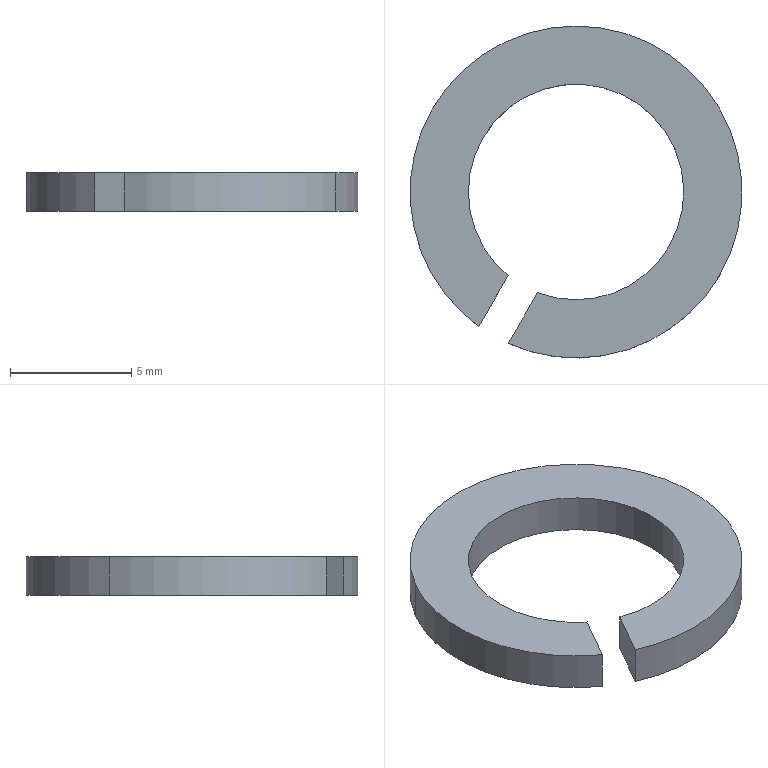Component | NX | SADDLE_SPRING_WASHER_8_4 | 1 solid | 10 faces | box 13.68 x 13.68 x 1.6 mm | volume 131 mm3 | cylinder 6 | plane 4 | commonest cylinder face diameters 8.88 x3 13.68 x3
STEP:
#1=CARTESIAN_POINT('',(0.,0.,0.));
#2=DIRECTION('',(0.,0.,1.));
#3=DIRECTION('',(1.,0.,0.));
#4=AXIS2_PLACEMENT_3D('',#1,#2,#3);
#5=CARTESIAN_POINT('',(-101.706,67.22,-42.5));
#6=VERTEX_POINT('',#5);
#7=CARTESIAN_POINT('',(-101.706,67.22,-40.9));
#8=VERTEX_POINT('',#7);
#9=CARTESIAN_POINT('',(-101.706,67.22,-41.7));
#10=DIRECTION('',(0.,0.,1.));
#11=VECTOR('',#10,1.);
#12=LINE('',#9,#11);
#13=CARTESIAN_POINT('',(-97.861,65.,-41.7));
#14=DIRECTION('',(0.,0.,1.));
#15=DIRECTION('',(0.866,-0.5,0.));
#16=AXIS2_PLACEMENT_3D('',#13,#14,#15);
#17=CYLINDRICAL_SURFACE('',#16,4.44);
#18=CARTESIAN_POINT('',(3.142,0.));
#19=DIRECTION('',(0.,1.));
#20=VECTOR('',#19,1.);
#21=LINE('',#18,#20);
#22=(GEOMETRIC_REPRESENTATION_CONTEXT(2)PARAMETRIC_REPRESENTATION_CONTEXT()REPRESENTATION_CONTEXT('',''));
#23=DEFINITIONAL_REPRESENTATION('',(#21),#22);
#24=PCURVE('',#17,#23);
#25=CARTESIAN_POINT('',(-97.861,65.,-41.7));
#26=DIRECTION('',(0.,0.,1.));
#27=DIRECTION('',(0.866,-0.5,0.));
#28=AXIS2_PLACEMENT_3D('',#25,#26,#27);
#29=CYLINDRICAL_SURFACE('',#28,4.44);
#30=CARTESIAN_POINT('',(3.142,0.));
#31=DIRECTION('',(0.,1.));
#32=VECTOR('',#31,1.);
#33=LINE('',#30,#32);
#34=(GEOMETRIC_REPRESENTATION_CONTEXT(2)PARAMETRIC_REPRESENTATION_CONTEXT()REPRESENTATION_CONTEXT('',''));
#35=DEFINITIONAL_REPRESENTATION('',(#33),#34);
#36=PCURVE('',#29,#35);
#37=SURFACE_CURVE('',#12,(#24,#36),.PCURVE_S1.);
#38=EDGE_CURVE('',#6,#8,#37,.T.);
#39=ORIENTED_EDGE('',*,*,#38,.T.);
#40=CARTESIAN_POINT('',(-94.016,62.78,-40.9));
#41=VERTEX_POINT('',#40);
#42=CARTESIAN_POINT('',(-97.861,65.,-40.9));
#43=DIRECTION('',(0.,0.,1.));
#44=DIRECTION('',(-0.866,0.5,0.));
#45=AXIS2_PLACEMENT_3D('',#42,#43,#44);
#46=CIRCLE('',#45,4.44);
#47=CARTESIAN_POINT('',(-3.142,0.8));
#48=DIRECTION('',(1.,0.));
#49=VECTOR('',#48,1.);
#50=LINE('',#47,#49);
#51=(GEOMETRIC_REPRESENTATION_CONTEXT(2)PARAMETRIC_REPRESENTATION_CONTEXT()REPRESENTATION_CONTEXT('',''));
#52=DEFINITIONAL_REPRESENTATION('',(#50),#51);
#53=PCURVE('',#17,#52);
#54=CARTESIAN_POINT('',(-97.861,65.,-40.9));
#55=DIRECTION('',(0.,0.,1.));
#56=DIRECTION('',(0.866,-0.5,0.));
#57=AXIS2_PLACEMENT_3D('',#54,#55,#56);
#58=PLANE('',#57);
#59=CARTESIAN_POINT('',(0.,0.));
#60=DIRECTION('',(-1.,0.));
#61=AXIS2_PLACEMENT_2D('',#59,#60);
#62=CIRCLE('',#61,4.44);
#63=(GEOMETRIC_REPRESENTATION_CONTEXT(2)PARAMETRIC_REPRESENTATION_CONTEXT()REPRESENTATION_CONTEXT('',''));
#64=DEFINITIONAL_REPRESENTATION('',(#62),#63);
#65=PCURVE('',#58,#64);
#66=SURFACE_CURVE('',#46,(#53,#65),.PCURVE_S1.);
#67=EDGE_CURVE('',#41,#8,#66,.T.);
#68=ORIENTED_EDGE('',*,*,#67,.F.);
#69=CARTESIAN_POINT('',(-94.016,62.78,-42.5));
#70=VERTEX_POINT('',#69);
#71=CARTESIAN_POINT('',(-94.016,62.78,-41.7));
#72=DIRECTION('',(0.,0.,1.));
#73=VECTOR('',#72,1.);
#74=LINE('',#71,#73);
#75=CARTESIAN_POINT('',(0.,0.));
#76=DIRECTION('',(0.,1.));
#77=VECTOR('',#76,1.);
#78=LINE('',#75,#77);
#79=(GEOMETRIC_REPRESENTATION_CONTEXT(2)PARAMETRIC_REPRESENTATION_CONTEXT()REPRESENTATION_CONTEXT('',''));
#80=DEFINITIONAL_REPRESENTATION('',(#78),#79);
#81=PCURVE('',#17,#80);
#82=CARTESIAN_POINT('',(-97.861,65.,-41.7));
#83=DIRECTION('',(0.,0.,1.));
#84=DIRECTION('',(0.866,-0.5,0.));
#85=AXIS2_PLACEMENT_3D('',#82,#83,#84);
#86=CYLINDRICAL_SURFACE('',#85,4.44);
#87=CARTESIAN_POINT('',(6.283,0.));
#88=DIRECTION('',(0.,1.));
#89=VECTOR('',#88,1.);
#90=LINE('',#87,#89);
#91=(GEOMETRIC_REPRESENTATION_CONTEXT(2)PARAMETRIC_REPRESENTATION_CONTEXT()REPRESENTATION_CONTEXT('',''));
#92=DEFINITIONAL_REPRESENTATION('',(#90),#91);
#93=PCURVE('',#86,#92);
#94=SURFACE_CURVE('',#74,(#81,#93),.PCURVE_S1.);
#95=EDGE_CURVE('',#70,#41,#94,.T.);
#96=ORIENTED_EDGE('',*,*,#95,.F.);
#97=CARTESIAN_POINT('',(-97.861,65.,-42.5));
#98=DIRECTION('',(0.,0.,1.));
#99=DIRECTION('',(-0.866,0.5,0.));
#100=AXIS2_PLACEMENT_3D('',#97,#98,#99);
#101=CIRCLE('',#100,4.44);
#102=CARTESIAN_POINT('',(-3.142,-0.8));
#103=DIRECTION('',(1.,0.));
#104=VECTOR('',#103,1.);
#105=LINE('',#102,#104);
#106=(GEOMETRIC_REPRESENTATION_CONTEXT(2)PARAMETRIC_REPRESENTATION_CONTEXT()REPRESENTATION_CONTEXT('',''));
#107=DEFINITIONAL_REPRESENTATION('',(#105),#106);
#108=PCURVE('',#17,#107);
#109=CARTESIAN_POINT('',(-97.861,65.,-42.5));
#110=DIRECTION('',(0.,0.,1.));
#111=DIRECTION('',(0.866,-0.5,0.));
#112=AXIS2_PLACEMENT_3D('',#109,#110,#111);
#113=PLANE('',#112);
#114=CARTESIAN_POINT('',(0.,0.));
#115=DIRECTION('',(-1.,0.));
#116=AXIS2_PLACEMENT_2D('',#114,#115);
#117=CIRCLE('',#116,4.44);
#118=(GEOMETRIC_REPRESENTATION_CONTEXT(2)PARAMETRIC_REPRESENTATION_CONTEXT()REPRESENTATION_CONTEXT('',''));
#119=DEFINITIONAL_REPRESENTATION('',(#117),#118);
#120=PCURVE('',#113,#119);
#121=SURFACE_CURVE('',#101,(#108,#120),.PCURVE_S1.);
#122=EDGE_CURVE('',#70,#6,#121,.T.);
#123=ORIENTED_EDGE('',*,*,#122,.T.);
#124=EDGE_LOOP('',(#39,#68,#96,#123));
#125=FACE_BOUND('',#124,.F.);
#126=ADVANCED_FACE('',(#125),#17,.F.);
#127=CARTESIAN_POINT('',(-100.659,61.553,-40.9));
#128=VERTEX_POINT('',#127);
#129=CARTESIAN_POINT('',(-100.659,61.553,-42.5));
#130=VERTEX_POINT('',#129);
#131=CARTESIAN_POINT('',(-100.659,61.553,-41.7));
#132=DIRECTION('',(0.,0.,-1.));
#133=VECTOR('',#132,1.);
#134=LINE('',#131,#133);
#135=CARTESIAN_POINT('',(4.554,0.));
#136=DIRECTION('',(0.,-1.));
#137=VECTOR('',#136,1.);
#138=LINE('',#135,#137);
#139=(GEOMETRIC_REPRESENTATION_CONTEXT(2)PARAMETRIC_REPRESENTATION_CONTEXT()REPRESENTATION_CONTEXT('',''));
#140=DEFINITIONAL_REPRESENTATION('',(#138),#139);
#141=PCURVE('',#29,#140);
#142=CARTESIAN_POINT('',(-100.609,61.641,-40.9));
#143=DIRECTION('',(-0.866,0.5,0.));
#144=DIRECTION('',(-0.5,-0.866,0.));
#145=AXIS2_PLACEMENT_3D('',#142,#143,#144);
#146=PLANE('',#145);
#147=CARTESIAN_POINT('',(0.1013,-0.8));
#148=DIRECTION('',(0.,-1.));
#149=VECTOR('',#148,1.);
#150=LINE('',#147,#149);
#151=(GEOMETRIC_REPRESENTATION_CONTEXT(2)PARAMETRIC_REPRESENTATION_CONTEXT()REPRESENTATION_CONTEXT('',''));
#152=DEFINITIONAL_REPRESENTATION('',(#150),#151);
#153=PCURVE('',#146,#152);
#154=SURFACE_CURVE('',#134,(#141,#153),.PCURVE_S1.);
#155=EDGE_CURVE('',#128,#130,#154,.T.);
#156=ORIENTED_EDGE('',*,*,#155,.F.);
#157=CARTESIAN_POINT('',(-97.861,65.,-40.9));
#158=DIRECTION('',(0.,0.,1.));
#159=DIRECTION('',(-0.866,0.5,0.));
#160=AXIS2_PLACEMENT_3D('',#157,#158,#159);
#161=CIRCLE('',#160,4.44);
#162=CARTESIAN_POINT('',(3.142,0.8));
#163=DIRECTION('',(1.,0.));
#164=VECTOR('',#163,1.);
#165=LINE('',#162,#164);
#166=(GEOMETRIC_REPRESENTATION_CONTEXT(2)PARAMETRIC_REPRESENTATION_CONTEXT()REPRESENTATION_CONTEXT('',''));
#167=DEFINITIONAL_REPRESENTATION('',(#165),#166);
#168=PCURVE('',#29,#167);
#169=CARTESIAN_POINT('',(0.,0.));
#170=DIRECTION('',(-1.,0.));
#171=AXIS2_PLACEMENT_2D('',#169,#170);
#172=CIRCLE('',#171,4.44);
#173=(GEOMETRIC_REPRESENTATION_CONTEXT(2)PARAMETRIC_REPRESENTATION_CONTEXT()REPRESENTATION_CONTEXT('',''));
#174=DEFINITIONAL_REPRESENTATION('',(#172),#173);
#175=PCURVE('',#58,#174);
#176=SURFACE_CURVE('',#161,(#168,#175),.PCURVE_S1.);
#177=EDGE_CURVE('',#8,#128,#176,.T.);
#178=ORIENTED_EDGE('',*,*,#177,.F.);
#179=ORIENTED_EDGE('',*,*,#38,.F.);
#180=CARTESIAN_POINT('',(-97.861,65.,-42.5));
#181=DIRECTION('',(0.,0.,1.));
#182=DIRECTION('',(-0.866,0.5,0.));
#183=AXIS2_PLACEMENT_3D('',#180,#181,#182);
#184=CIRCLE('',#183,4.44);
#185=CARTESIAN_POINT('',(3.142,-0.8));
#186=DIRECTION('',(1.,0.));
#187=VECTOR('',#186,1.);
#188=LINE('',#185,#187);
#189=(GEOMETRIC_REPRESENTATION_CONTEXT(2)PARAMETRIC_REPRESENTATION_CONTEXT()REPRESENTATION_CONTEXT('',''));
#190=DEFINITIONAL_REPRESENTATION('',(#188),#189);
#191=PCURVE('',#29,#190);
#192=CARTESIAN_POINT('',(0.,0.));
#193=DIRECTION('',(-1.,0.));
#194=AXIS2_PLACEMENT_2D('',#192,#193);
#195=CIRCLE('',#194,4.44);
#196=(GEOMETRIC_REPRESENTATION_CONTEXT(2)PARAMETRIC_REPRESENTATION_CONTEXT()REPRESENTATION_CONTEXT('',''));
#197=DEFINITIONAL_REPRESENTATION('',(#195),#196);
#198=PCURVE('',#113,#197);
#199=SURFACE_CURVE('',#184,(#191,#198),.PCURVE_S1.);
#200=EDGE_CURVE('',#6,#130,#199,.T.);
#201=ORIENTED_EDGE('',*,*,#200,.T.);
#202=EDGE_LOOP('',(#156,#178,#179,#201));
#203=FACE_BOUND('',#202,.F.);
#204=ADVANCED_FACE('',(#203),#29,.F.);
#205=CARTESIAN_POINT('',(-100.657,58.757,-42.5));
#206=VERTEX_POINT('',#205);
#207=CARTESIAN_POINT('',(-91.937,61.58,-42.5));
#208=VERTEX_POINT('',#207);
#209=CARTESIAN_POINT('',(-97.861,65.,-42.5));
#210=DIRECTION('',(0.,0.,1.));
#211=DIRECTION('',(-0.866,0.5,0.));
#212=AXIS2_PLACEMENT_3D('',#209,#210,#211);
#213=CIRCLE('',#212,6.84);
#214=CARTESIAN_POINT('',(-97.861,65.,-41.7));
#215=DIRECTION('',(0.,0.,1.));
#216=DIRECTION('',(0.866,-0.5,0.));
#217=AXIS2_PLACEMENT_3D('',#214,#215,#216);
#218=CYLINDRICAL_SURFACE('',#217,6.84);
#219=CARTESIAN_POINT('',(3.142,-0.8));
#220=DIRECTION('',(1.,0.));
#221=VECTOR('',#220,1.);
#222=LINE('',#219,#221);
#223=(GEOMETRIC_REPRESENTATION_CONTEXT(2)PARAMETRIC_REPRESENTATION_CONTEXT()REPRESENTATION_CONTEXT('',''));
#224=DEFINITIONAL_REPRESENTATION('',(#222),#223);
#225=PCURVE('',#218,#224);
#226=CARTESIAN_POINT('',(0.,0.));
#227=DIRECTION('',(-1.,0.));
#228=AXIS2_PLACEMENT_2D('',#226,#227);
#229=CIRCLE('',#228,6.84);
#230=(GEOMETRIC_REPRESENTATION_CONTEXT(2)PARAMETRIC_REPRESENTATION_CONTEXT()REPRESENTATION_CONTEXT('',''));
#231=DEFINITIONAL_REPRESENTATION('',(#229),#230);
#232=PCURVE('',#113,#231);
#233=SURFACE_CURVE('',#213,(#225,#232),.PCURVE_S1.);
#234=EDGE_CURVE('',#206,#208,#233,.T.);
#235=ORIENTED_EDGE('',*,*,#234,.T.);
#236=CARTESIAN_POINT('',(-91.937,61.58,-40.9));
#237=VERTEX_POINT('',#236);
#238=CARTESIAN_POINT('',(-91.937,61.58,-41.7));
#239=DIRECTION('',(0.,0.,1.));
#240=VECTOR('',#239,1.);
#241=LINE('',#238,#240);
#242=CARTESIAN_POINT('',(6.283,0.));
#243=DIRECTION('',(0.,1.));
#244=VECTOR('',#243,1.);
#245=LINE('',#242,#244);
#246=(GEOMETRIC_REPRESENTATION_CONTEXT(2)PARAMETRIC_REPRESENTATION_CONTEXT()REPRESENTATION_CONTEXT('',''));
#247=DEFINITIONAL_REPRESENTATION('',(#245),#246);
#248=PCURVE('',#218,#247);
#249=CARTESIAN_POINT('',(-97.861,65.,-41.7));
#250=DIRECTION('',(0.,0.,1.));
#251=DIRECTION('',(0.866,-0.5,0.));
#252=AXIS2_PLACEMENT_3D('',#249,#250,#251);
#253=CYLINDRICAL_SURFACE('',#252,6.84);
#254=CARTESIAN_POINT('',(0.,0.));
#255=DIRECTION('',(0.,1.));
#256=VECTOR('',#255,1.);
#257=LINE('',#254,#256);
#258=(GEOMETRIC_REPRESENTATION_CONTEXT(2)PARAMETRIC_REPRESENTATION_CONTEXT()REPRESENTATION_CONTEXT('',''));
#259=DEFINITIONAL_REPRESENTATION('',(#257),#258);
#260=PCURVE('',#253,#259);
#261=SURFACE_CURVE('',#241,(#248,#260),.PCURVE_S1.);
#262=EDGE_CURVE('',#208,#237,#261,.T.);
#263=ORIENTED_EDGE('',*,*,#262,.T.);
#264=CARTESIAN_POINT('',(-100.657,58.757,-40.9));
#265=VERTEX_POINT('',#264);
#266=CARTESIAN_POINT('',(-97.861,65.,-40.9));
#267=DIRECTION('',(0.,0.,1.));
#268=DIRECTION('',(-0.866,0.5,0.));
#269=AXIS2_PLACEMENT_3D('',#266,#267,#268);
#270=CIRCLE('',#269,6.84);
#271=CARTESIAN_POINT('',(3.142,0.8));
#272=DIRECTION('',(1.,0.));
#273=VECTOR('',#272,1.);
#274=LINE('',#271,#273);
#275=(GEOMETRIC_REPRESENTATION_CONTEXT(2)PARAMETRIC_REPRESENTATION_CONTEXT()REPRESENTATION_CONTEXT('',''));
#276=DEFINITIONAL_REPRESENTATION('',(#274),#275);
#277=PCURVE('',#218,#276);
#278=CARTESIAN_POINT('',(0.,0.));
#279=DIRECTION('',(-1.,0.));
#280=AXIS2_PLACEMENT_2D('',#278,#279);
#281=CIRCLE('',#280,6.84);
#282=(GEOMETRIC_REPRESENTATION_CONTEXT(2)PARAMETRIC_REPRESENTATION_CONTEXT()REPRESENTATION_CONTEXT('',''));
#283=DEFINITIONAL_REPRESENTATION('',(#281),#282);
#284=PCURVE('',#58,#283);
#285=SURFACE_CURVE('',#270,(#277,#284),.PCURVE_S1.);
#286=EDGE_CURVE('',#265,#237,#285,.T.);
#287=ORIENTED_EDGE('',*,*,#286,.F.);
#288=CARTESIAN_POINT('',(-100.657,58.757,-41.7));
#289=DIRECTION('',(0.,0.,-1.));
#290=VECTOR('',#289,1.);
#291=LINE('',#288,#290);
#292=CARTESIAN_POINT('',(4.815,0.));
#293=DIRECTION('',(0.,-1.));
#294=VECTOR('',#293,1.);
#295=LINE('',#292,#294);
#296=(GEOMETRIC_REPRESENTATION_CONTEXT(2)PARAMETRIC_REPRESENTATION_CONTEXT()REPRESENTATION_CONTEXT('',''));
#297=DEFINITIONAL_REPRESENTATION('',(#295),#296);
#298=PCURVE('',#218,#297);
#299=CARTESIAN_POINT('',(-99.396,60.941,-40.9));
#300=DIRECTION('',(0.866,-0.5,0.));
#301=DIRECTION('',(0.5,0.866,0.));
#302=AXIS2_PLACEMENT_3D('',#299,#300,#301);
#303=PLANE('',#302);
#304=CARTESIAN_POINT('',(-2.521,-0.8));
#305=DIRECTION('',(0.,-1.));
#306=VECTOR('',#305,1.);
#307=LINE('',#304,#306);
#308=(GEOMETRIC_REPRESENTATION_CONTEXT(2)PARAMETRIC_REPRESENTATION_CONTEXT()REPRESENTATION_CONTEXT('',''));
#309=DEFINITIONAL_REPRESENTATION('',(#307),#308);
#310=PCURVE('',#303,#309);
#311=SURFACE_CURVE('',#291,(#298,#310),.PCURVE_S1.);
#312=EDGE_CURVE('',#265,#206,#311,.T.);
#313=ORIENTED_EDGE('',*,*,#312,.T.);
#314=EDGE_LOOP('',(#235,#263,#287,#313));
#315=FACE_BOUND('',#314,.T.);
#316=ADVANCED_FACE('',(#315),#218,.T.);
#317=ORIENTED_EDGE('',*,*,#262,.F.);
#318=CARTESIAN_POINT('',(-103.784,68.42,-42.5));
#319=VERTEX_POINT('',#318);
#320=CARTESIAN_POINT('',(-97.861,65.,-42.5));
#321=DIRECTION('',(0.,0.,1.));
#322=DIRECTION('',(-0.866,0.5,0.));
#323=AXIS2_PLACEMENT_3D('',#320,#321,#322);
#324=CIRCLE('',#323,6.84);
#325=CARTESIAN_POINT('',(-3.142,-0.8));
#326=DIRECTION('',(1.,0.));
#327=VECTOR('',#326,1.);
#328=LINE('',#325,#327);
#329=(GEOMETRIC_REPRESENTATION_CONTEXT(2)PARAMETRIC_REPRESENTATION_CONTEXT()REPRESENTATION_CONTEXT('',''));
#330=DEFINITIONAL_REPRESENTATION('',(#328),#329);
#331=PCURVE('',#253,#330);
#332=CARTESIAN_POINT('',(0.,0.));
#333=DIRECTION('',(-1.,0.));
#334=AXIS2_PLACEMENT_2D('',#332,#333);
#335=CIRCLE('',#334,6.84);
#336=(GEOMETRIC_REPRESENTATION_CONTEXT(2)PARAMETRIC_REPRESENTATION_CONTEXT()REPRESENTATION_CONTEXT('',''));
#337=DEFINITIONAL_REPRESENTATION('',(#335),#336);
#338=PCURVE('',#113,#337);
#339=SURFACE_CURVE('',#324,(#331,#338),.PCURVE_S1.);
#340=EDGE_CURVE('',#208,#319,#339,.T.);
#341=ORIENTED_EDGE('',*,*,#340,.T.);
#342=CARTESIAN_POINT('',(-103.784,68.42,-40.9));
#343=VERTEX_POINT('',#342);
#344=CARTESIAN_POINT('',(-103.784,68.42,-41.7));
#345=DIRECTION('',(0.,0.,1.));
#346=VECTOR('',#345,1.);
#347=LINE('',#344,#346);
#348=CARTESIAN_POINT('',(3.142,0.));
#349=DIRECTION('',(0.,1.));
#350=VECTOR('',#349,1.);
#351=LINE('',#348,#350);
#352=(GEOMETRIC_REPRESENTATION_CONTEXT(2)PARAMETRIC_REPRESENTATION_CONTEXT()REPRESENTATION_CONTEXT('',''));
#353=DEFINITIONAL_REPRESENTATION('',(#351),#352);
#354=PCURVE('',#253,#353);
#355=CARTESIAN_POINT('',(-97.861,65.,-41.7));
#356=DIRECTION('',(0.,0.,1.));
#357=DIRECTION('',(0.866,-0.5,0.));
#358=AXIS2_PLACEMENT_3D('',#355,#356,#357);
#359=CYLINDRICAL_SURFACE('',#358,6.84);
#360=CARTESIAN_POINT('',(3.142,0.));
#361=DIRECTION('',(0.,1.));
#362=VECTOR('',#361,1.);
#363=LINE('',#360,#362);
#364=(GEOMETRIC_REPRESENTATION_CONTEXT(2)PARAMETRIC_REPRESENTATION_CONTEXT()REPRESENTATION_CONTEXT('',''));
#365=DEFINITIONAL_REPRESENTATION('',(#363),#364);
#366=PCURVE('',#359,#365);
#367=SURFACE_CURVE('',#347,(#354,#366),.PCURVE_S1.);
#368=EDGE_CURVE('',#319,#343,#367,.T.);
#369=ORIENTED_EDGE('',*,*,#368,.T.);
#370=CARTESIAN_POINT('',(-97.861,65.,-40.9));
#371=DIRECTION('',(0.,0.,1.));
#372=DIRECTION('',(-0.866,0.5,0.));
#373=AXIS2_PLACEMENT_3D('',#370,#371,#372);
#374=CIRCLE('',#373,6.84);
#375=CARTESIAN_POINT('',(-3.142,0.8));
#376=DIRECTION('',(1.,0.));
#377=VECTOR('',#376,1.);
#378=LINE('',#375,#377);
#379=(GEOMETRIC_REPRESENTATION_CONTEXT(2)PARAMETRIC_REPRESENTATION_CONTEXT()REPRESENTATION_CONTEXT('',''));
#380=DEFINITIONAL_REPRESENTATION('',(#378),#379);
#381=PCURVE('',#253,#380);
#382=CARTESIAN_POINT('',(0.,0.));
#383=DIRECTION('',(-1.,0.));
#384=AXIS2_PLACEMENT_2D('',#382,#383);
#385=CIRCLE('',#384,6.84);
#386=(GEOMETRIC_REPRESENTATION_CONTEXT(2)PARAMETRIC_REPRESENTATION_CONTEXT()REPRESENTATION_CONTEXT('',''));
#387=DEFINITIONAL_REPRESENTATION('',(#385),#386);
#388=PCURVE('',#58,#387);
#389=SURFACE_CURVE('',#374,(#381,#388),.PCURVE_S1.);
#390=EDGE_CURVE('',#237,#343,#389,.T.);
#391=ORIENTED_EDGE('',*,*,#390,.F.);
#392=EDGE_LOOP('',(#317,#341,#369,#391));
#393=FACE_BOUND('',#392,.T.);
#394=ADVANCED_FACE('',(#393),#253,.T.);
#395=ORIENTED_EDGE('',*,*,#368,.F.);
#396=CARTESIAN_POINT('',(-101.869,59.457,-42.5));
#397=VERTEX_POINT('',#396);
#398=CARTESIAN_POINT('',(-97.861,65.,-42.5));
#399=DIRECTION('',(0.,0.,1.));
#400=DIRECTION('',(-0.866,0.5,0.));
#401=AXIS2_PLACEMENT_3D('',#398,#399,#400);
#402=CIRCLE('',#401,6.84);
#403=CARTESIAN_POINT('',(3.142,-0.8));
#404=DIRECTION('',(1.,0.));
#405=VECTOR('',#404,1.);
#406=LINE('',#403,#405);
#407=(GEOMETRIC_REPRESENTATION_CONTEXT(2)PARAMETRIC_REPRESENTATION_CONTEXT()REPRESENTATION_CONTEXT('',''));
#408=DEFINITIONAL_REPRESENTATION('',(#406),#407);
#409=PCURVE('',#359,#408);
#410=CARTESIAN_POINT('',(0.,0.));
#411=DIRECTION('',(-1.,0.));
#412=AXIS2_PLACEMENT_2D('',#410,#411);
#413=CIRCLE('',#412,6.84);
#414=(GEOMETRIC_REPRESENTATION_CONTEXT(2)PARAMETRIC_REPRESENTATION_CONTEXT()REPRESENTATION_CONTEXT('',''));
#415=DEFINITIONAL_REPRESENTATION('',(#413),#414);
#416=PCURVE('',#113,#415);
#417=SURFACE_CURVE('',#402,(#409,#416),.PCURVE_S1.);
#418=EDGE_CURVE('',#319,#397,#417,.T.);
#419=ORIENTED_EDGE('',*,*,#418,.T.);
#420=CARTESIAN_POINT('',(-101.869,59.457,-40.9));
#421=VERTEX_POINT('',#420);
#422=CARTESIAN_POINT('',(-101.869,59.457,-41.7));
#423=DIRECTION('',(0.,0.,1.));
#424=VECTOR('',#423,1.);
#425=LINE('',#422,#424);
#426=CARTESIAN_POINT('',(4.61,0.));
#427=DIRECTION('',(0.,1.));
#428=VECTOR('',#427,1.);
#429=LINE('',#426,#428);
#430=(GEOMETRIC_REPRESENTATION_CONTEXT(2)PARAMETRIC_REPRESENTATION_CONTEXT()REPRESENTATION_CONTEXT('',''));
#431=DEFINITIONAL_REPRESENTATION('',(#429),#430);
#432=PCURVE('',#359,#431);
#433=CARTESIAN_POINT('',(2.521,-0.8));
#434=DIRECTION('',(0.,1.));
#435=VECTOR('',#434,1.);
#436=LINE('',#433,#435);
#437=(GEOMETRIC_REPRESENTATION_CONTEXT(2)PARAMETRIC_REPRESENTATION_CONTEXT()REPRESENTATION_CONTEXT('',''));
#438=DEFINITIONAL_REPRESENTATION('',(#436),#437);
#439=PCURVE('',#146,#438);
#440=SURFACE_CURVE('',#425,(#432,#439),.PCURVE_S1.);
#441=EDGE_CURVE('',#397,#421,#440,.T.);
#442=ORIENTED_EDGE('',*,*,#441,.T.);
#443=CARTESIAN_POINT('',(-97.861,65.,-40.9));
#444=DIRECTION('',(0.,0.,1.));
#445=DIRECTION('',(-0.866,0.5,0.));
#446=AXIS2_PLACEMENT_3D('',#443,#444,#445);
#447=CIRCLE('',#446,6.84);
#448=CARTESIAN_POINT('',(3.142,0.8));
#449=DIRECTION('',(1.,0.));
#450=VECTOR('',#449,1.);
#451=LINE('',#448,#450);
#452=(GEOMETRIC_REPRESENTATION_CONTEXT(2)PARAMETRIC_REPRESENTATION_CONTEXT()REPRESENTATION_CONTEXT('',''));
#453=DEFINITIONAL_REPRESENTATION('',(#451),#452);
#454=PCURVE('',#359,#453);
#455=CARTESIAN_POINT('',(0.,0.));
#456=DIRECTION('',(-1.,0.));
#457=AXIS2_PLACEMENT_2D('',#455,#456);
#458=CIRCLE('',#457,6.84);
#459=(GEOMETRIC_REPRESENTATION_CONTEXT(2)PARAMETRIC_REPRESENTATION_CONTEXT()REPRESENTATION_CONTEXT('',''));
#460=DEFINITIONAL_REPRESENTATION('',(#458),#459);
#461=PCURVE('',#58,#460);
#462=SURFACE_CURVE('',#447,(#454,#461),.PCURVE_S1.);
#463=EDGE_CURVE('',#343,#421,#462,.T.);
#464=ORIENTED_EDGE('',*,*,#463,.F.);
#465=EDGE_LOOP('',(#395,#419,#442,#464));
#466=FACE_BOUND('',#465,.T.);
#467=ADVANCED_FACE('',(#466),#359,.T.);
#468=CARTESIAN_POINT('',(-99.447,60.853,-42.5));
#469=VERTEX_POINT('',#468);
#470=CARTESIAN_POINT('',(-97.861,65.,-42.5));
#471=DIRECTION('',(0.,0.,1.));
#472=DIRECTION('',(-0.866,0.5,0.));
#473=AXIS2_PLACEMENT_3D('',#470,#471,#472);
#474=CIRCLE('',#473,4.44);
#475=CARTESIAN_POINT('',(0.,0.));
#476=DIRECTION('',(-1.,0.));
#477=AXIS2_PLACEMENT_2D('',#475,#476);
#478=CIRCLE('',#477,4.44);
#479=(GEOMETRIC_REPRESENTATION_CONTEXT(2)PARAMETRIC_REPRESENTATION_CONTEXT()REPRESENTATION_CONTEXT('',''));
#480=DEFINITIONAL_REPRESENTATION('',(#478),#479);
#481=PCURVE('',#113,#480);
#482=CARTESIAN_POINT('',(3.142,-0.8));
#483=DIRECTION('',(1.,0.));
#484=VECTOR('',#483,1.);
#485=LINE('',#482,#484);
#486=(GEOMETRIC_REPRESENTATION_CONTEXT(2)PARAMETRIC_REPRESENTATION_CONTEXT()REPRESENTATION_CONTEXT('',''));
#487=DEFINITIONAL_REPRESENTATION('',(#485),#486);
#488=PCURVE('',#86,#487);
#489=SURFACE_CURVE('',#474,(#481,#488),.PCURVE_S1.);
#490=EDGE_CURVE('',#469,#70,#489,.T.);
#491=ORIENTED_EDGE('',*,*,#490,.T.);
#492=ORIENTED_EDGE('',*,*,#122,.T.);
#493=ORIENTED_EDGE('',*,*,#200,.T.);
#494=CARTESIAN_POINT('',(-100.609,61.641,-42.5));
#495=DIRECTION('',(0.5,0.866,0.));
#496=VECTOR('',#495,1.);
#497=LINE('',#494,#496);
#498=CARTESIAN_POINT('',(-0.7,-4.283));
#499=DIRECTION('',(0.,1.));
#500=VECTOR('',#499,1.);
#501=LINE('',#498,#500);
#502=(GEOMETRIC_REPRESENTATION_CONTEXT(2)PARAMETRIC_REPRESENTATION_CONTEXT()REPRESENTATION_CONTEXT('',''));
#503=DEFINITIONAL_REPRESENTATION('',(#501),#502);
#504=PCURVE('',#113,#503);
#505=CARTESIAN_POINT('',(0.,-1.6));
#506=DIRECTION('',(-1.,0.));
#507=VECTOR('',#506,1.);
#508=LINE('',#505,#507);
#509=(GEOMETRIC_REPRESENTATION_CONTEXT(2)PARAMETRIC_REPRESENTATION_CONTEXT()REPRESENTATION_CONTEXT('',''));
#510=DEFINITIONAL_REPRESENTATION('',(#508),#509);
#511=PCURVE('',#146,#510);
#512=SURFACE_CURVE('',#497,(#504,#511),.PCURVE_S1.);
#513=EDGE_CURVE('',#397,#130,#512,.T.);
#514=ORIENTED_EDGE('',*,*,#513,.F.);
#515=ORIENTED_EDGE('',*,*,#418,.F.);
#516=ORIENTED_EDGE('',*,*,#340,.F.);
#517=ORIENTED_EDGE('',*,*,#234,.F.);
#518=CARTESIAN_POINT('',(-99.396,60.941,-42.5));
#519=DIRECTION('',(-0.5,-0.866,0.));
#520=VECTOR('',#519,1.);
#521=LINE('',#518,#520);
#522=CARTESIAN_POINT('',(0.7,-4.283));
#523=DIRECTION('',(0.,-1.));
#524=VECTOR('',#523,1.);
#525=LINE('',#522,#524);
#526=(GEOMETRIC_REPRESENTATION_CONTEXT(2)PARAMETRIC_REPRESENTATION_CONTEXT()REPRESENTATION_CONTEXT('',''));
#527=DEFINITIONAL_REPRESENTATION('',(#525),#526);
#528=PCURVE('',#113,#527);
#529=CARTESIAN_POINT('',(0.,-1.6));
#530=DIRECTION('',(-1.,0.));
#531=VECTOR('',#530,1.);
#532=LINE('',#529,#531);
#533=(GEOMETRIC_REPRESENTATION_CONTEXT(2)PARAMETRIC_REPRESENTATION_CONTEXT()REPRESENTATION_CONTEXT('',''));
#534=DEFINITIONAL_REPRESENTATION('',(#532),#533);
#535=PCURVE('',#303,#534);
#536=SURFACE_CURVE('',#521,(#528,#535),.PCURVE_S1.);
#537=EDGE_CURVE('',#469,#206,#536,.T.);
#538=ORIENTED_EDGE('',*,*,#537,.F.);
#539=EDGE_LOOP('',(#491,#492,#493,#514,#515,#516,#517,#538));
#540=FACE_BOUND('',#539,.T.);
#541=ADVANCED_FACE('',(#540),#113,.F.);
#542=CARTESIAN_POINT('',(-99.447,60.853,-40.9));
#543=VERTEX_POINT('',#542);
#544=CARTESIAN_POINT('',(-97.861,65.,-40.9));
#545=DIRECTION('',(0.,0.,1.));
#546=DIRECTION('',(-0.866,0.5,0.));
#547=AXIS2_PLACEMENT_3D('',#544,#545,#546);
#548=CIRCLE('',#547,4.44);
#549=CARTESIAN_POINT('',(3.142,0.8));
#550=DIRECTION('',(1.,0.));
#551=VECTOR('',#550,1.);
#552=LINE('',#549,#551);
#553=(GEOMETRIC_REPRESENTATION_CONTEXT(2)PARAMETRIC_REPRESENTATION_CONTEXT()REPRESENTATION_CONTEXT('',''));
#554=DEFINITIONAL_REPRESENTATION('',(#552),#553);
#555=PCURVE('',#86,#554);
#556=CARTESIAN_POINT('',(0.,0.));
#557=DIRECTION('',(-1.,0.));
#558=AXIS2_PLACEMENT_2D('',#556,#557);
#559=CIRCLE('',#558,4.44);
#560=(GEOMETRIC_REPRESENTATION_CONTEXT(2)PARAMETRIC_REPRESENTATION_CONTEXT()REPRESENTATION_CONTEXT('',''));
#561=DEFINITIONAL_REPRESENTATION('',(#559),#560);
#562=PCURVE('',#58,#561);
#563=SURFACE_CURVE('',#548,(#555,#562),.PCURVE_S1.);
#564=EDGE_CURVE('',#543,#41,#563,.T.);
#565=ORIENTED_EDGE('',*,*,#564,.F.);
#566=CARTESIAN_POINT('',(-99.447,60.853,-41.7));
#567=DIRECTION('',(0.,0.,-1.));
#568=VECTOR('',#567,1.);
#569=LINE('',#566,#568);
#570=CARTESIAN_POINT('',(4.871,0.));
#571=DIRECTION('',(0.,-1.));
#572=VECTOR('',#571,1.);
#573=LINE('',#570,#572);
#574=(GEOMETRIC_REPRESENTATION_CONTEXT(2)PARAMETRIC_REPRESENTATION_CONTEXT()REPRESENTATION_CONTEXT('',''));
#575=DEFINITIONAL_REPRESENTATION('',(#573),#574);
#576=PCURVE('',#86,#575);
#577=CARTESIAN_POINT('',(-0.1013,-0.8));
#578=DIRECTION('',(0.,-1.));
#579=VECTOR('',#578,1.);
#580=LINE('',#577,#579);
#581=(GEOMETRIC_REPRESENTATION_CONTEXT(2)PARAMETRIC_REPRESENTATION_CONTEXT()REPRESENTATION_CONTEXT('',''));
#582=DEFINITIONAL_REPRESENTATION('',(#580),#581);
#583=PCURVE('',#303,#582);
#584=SURFACE_CURVE('',#569,(#576,#583),.PCURVE_S1.);
#585=EDGE_CURVE('',#543,#469,#584,.T.);
#586=ORIENTED_EDGE('',*,*,#585,.T.);
#587=ORIENTED_EDGE('',*,*,#490,.T.);
#588=ORIENTED_EDGE('',*,*,#95,.T.);
#589=EDGE_LOOP('',(#565,#586,#587,#588));
#590=FACE_BOUND('',#589,.F.);
#591=ADVANCED_FACE('',(#590),#86,.F.);
#592=CARTESIAN_POINT('',(-98.467,65.35,-40.9));
#593=DIRECTION('',(-0.5,-0.866,0.));
#594=VECTOR('',#593,1.);
#595=LINE('',#592,#594);
#596=CARTESIAN_POINT('',(-0.7,0.));
#597=DIRECTION('',(0.,-1.));
#598=VECTOR('',#597,1.);
#599=LINE('',#596,#598);
#600=(GEOMETRIC_REPRESENTATION_CONTEXT(2)PARAMETRIC_REPRESENTATION_CONTEXT()REPRESENTATION_CONTEXT('',''));
#601=DEFINITIONAL_REPRESENTATION('',(#599),#600);
#602=PCURVE('',#58,#601);
#603=CARTESIAN_POINT('',(-4.283,0.));
#604=DIRECTION('',(1.,0.));
#605=VECTOR('',#604,1.);
#606=LINE('',#603,#605);
#607=(GEOMETRIC_REPRESENTATION_CONTEXT(2)PARAMETRIC_REPRESENTATION_CONTEXT()REPRESENTATION_CONTEXT('',''));
#608=DEFINITIONAL_REPRESENTATION('',(#606),#607);
#609=PCURVE('',#146,#608);
#610=SURFACE_CURVE('',#595,(#602,#609),.PCURVE_S1.);
#611=EDGE_CURVE('',#128,#421,#610,.T.);
#612=ORIENTED_EDGE('',*,*,#611,.F.);
#613=ORIENTED_EDGE('',*,*,#177,.F.);
#614=ORIENTED_EDGE('',*,*,#67,.F.);
#615=ORIENTED_EDGE('',*,*,#564,.F.);
#616=CARTESIAN_POINT('',(-99.396,60.941,-40.9));
#617=DIRECTION('',(-0.5,-0.866,0.));
#618=VECTOR('',#617,1.);
#619=LINE('',#616,#618);
#620=CARTESIAN_POINT('',(0.7,-4.283));
#621=DIRECTION('',(0.,-1.));
#622=VECTOR('',#621,1.);
#623=LINE('',#620,#622);
#624=(GEOMETRIC_REPRESENTATION_CONTEXT(2)PARAMETRIC_REPRESENTATION_CONTEXT()REPRESENTATION_CONTEXT('',''));
#625=DEFINITIONAL_REPRESENTATION('',(#623),#624);
#626=PCURVE('',#58,#625);
#627=CARTESIAN_POINT('',(0.,0.));
#628=DIRECTION('',(-1.,0.));
#629=VECTOR('',#628,1.);
#630=LINE('',#627,#629);
#631=(GEOMETRIC_REPRESENTATION_CONTEXT(2)PARAMETRIC_REPRESENTATION_CONTEXT()REPRESENTATION_CONTEXT('',''));
#632=DEFINITIONAL_REPRESENTATION('',(#630),#631);
#633=PCURVE('',#303,#632);
#634=SURFACE_CURVE('',#619,(#626,#633),.PCURVE_S1.);
#635=EDGE_CURVE('',#543,#265,#634,.T.);
#636=ORIENTED_EDGE('',*,*,#635,.T.);
#637=ORIENTED_EDGE('',*,*,#286,.T.);
#638=ORIENTED_EDGE('',*,*,#390,.T.);
#639=ORIENTED_EDGE('',*,*,#463,.T.);
#640=EDGE_LOOP('',(#612,#613,#614,#615,#636,#637,#638,#639));
#641=FACE_BOUND('',#640,.T.);
#642=ADVANCED_FACE('',(#641),#58,.T.);
#643=ORIENTED_EDGE('',*,*,#635,.F.);
#644=ORIENTED_EDGE('',*,*,#585,.T.);
#645=ORIENTED_EDGE('',*,*,#537,.T.);
#646=ORIENTED_EDGE('',*,*,#312,.F.);
#647=EDGE_LOOP('',(#643,#644,#645,#646));
#648=FACE_BOUND('',#647,.T.);
#649=ADVANCED_FACE('',(#648),#303,.F.);
#650=ORIENTED_EDGE('',*,*,#513,.T.);
#651=ORIENTED_EDGE('',*,*,#155,.F.);
#652=ORIENTED_EDGE('',*,*,#611,.T.);
#653=ORIENTED_EDGE('',*,*,#441,.F.);
#654=EDGE_LOOP('',(#650,#651,#652,#653));
#655=FACE_BOUND('',#654,.T.);
#656=ADVANCED_FACE('',(#655),#146,.F.);
#657=CLOSED_SHELL('',(#126,#204,#316,#394,#467,#541,#591,#642,#649,#656));
#658=MANIFOLD_SOLID_BREP('',#657);
#659=(LENGTH_UNIT()NAMED_UNIT(*)SI_UNIT(.MILLI.,.METRE.));
#660=UNCERTAINTY_MEASURE_WITH_UNIT(LENGTH_MEASURE(0.0000001),#659,'','');
#661=(NAMED_UNIT(*)PLANE_ANGLE_UNIT()SI_UNIT($,.RADIAN.));
#662=(NAMED_UNIT(*)SI_UNIT($,.STERADIAN.)SOLID_ANGLE_UNIT());
#663=(GEOMETRIC_REPRESENTATION_CONTEXT(3)GLOBAL_UNCERTAINTY_ASSIGNED_CONTEXT((#660))GLOBAL_UNIT_ASSIGNED_CONTEXT((#659,#661,#662))REPRESENTATION_CONTEXT('',''));
#664=ADVANCED_BREP_SHAPE_REPRESENTATION('',(#4,#658),#663);